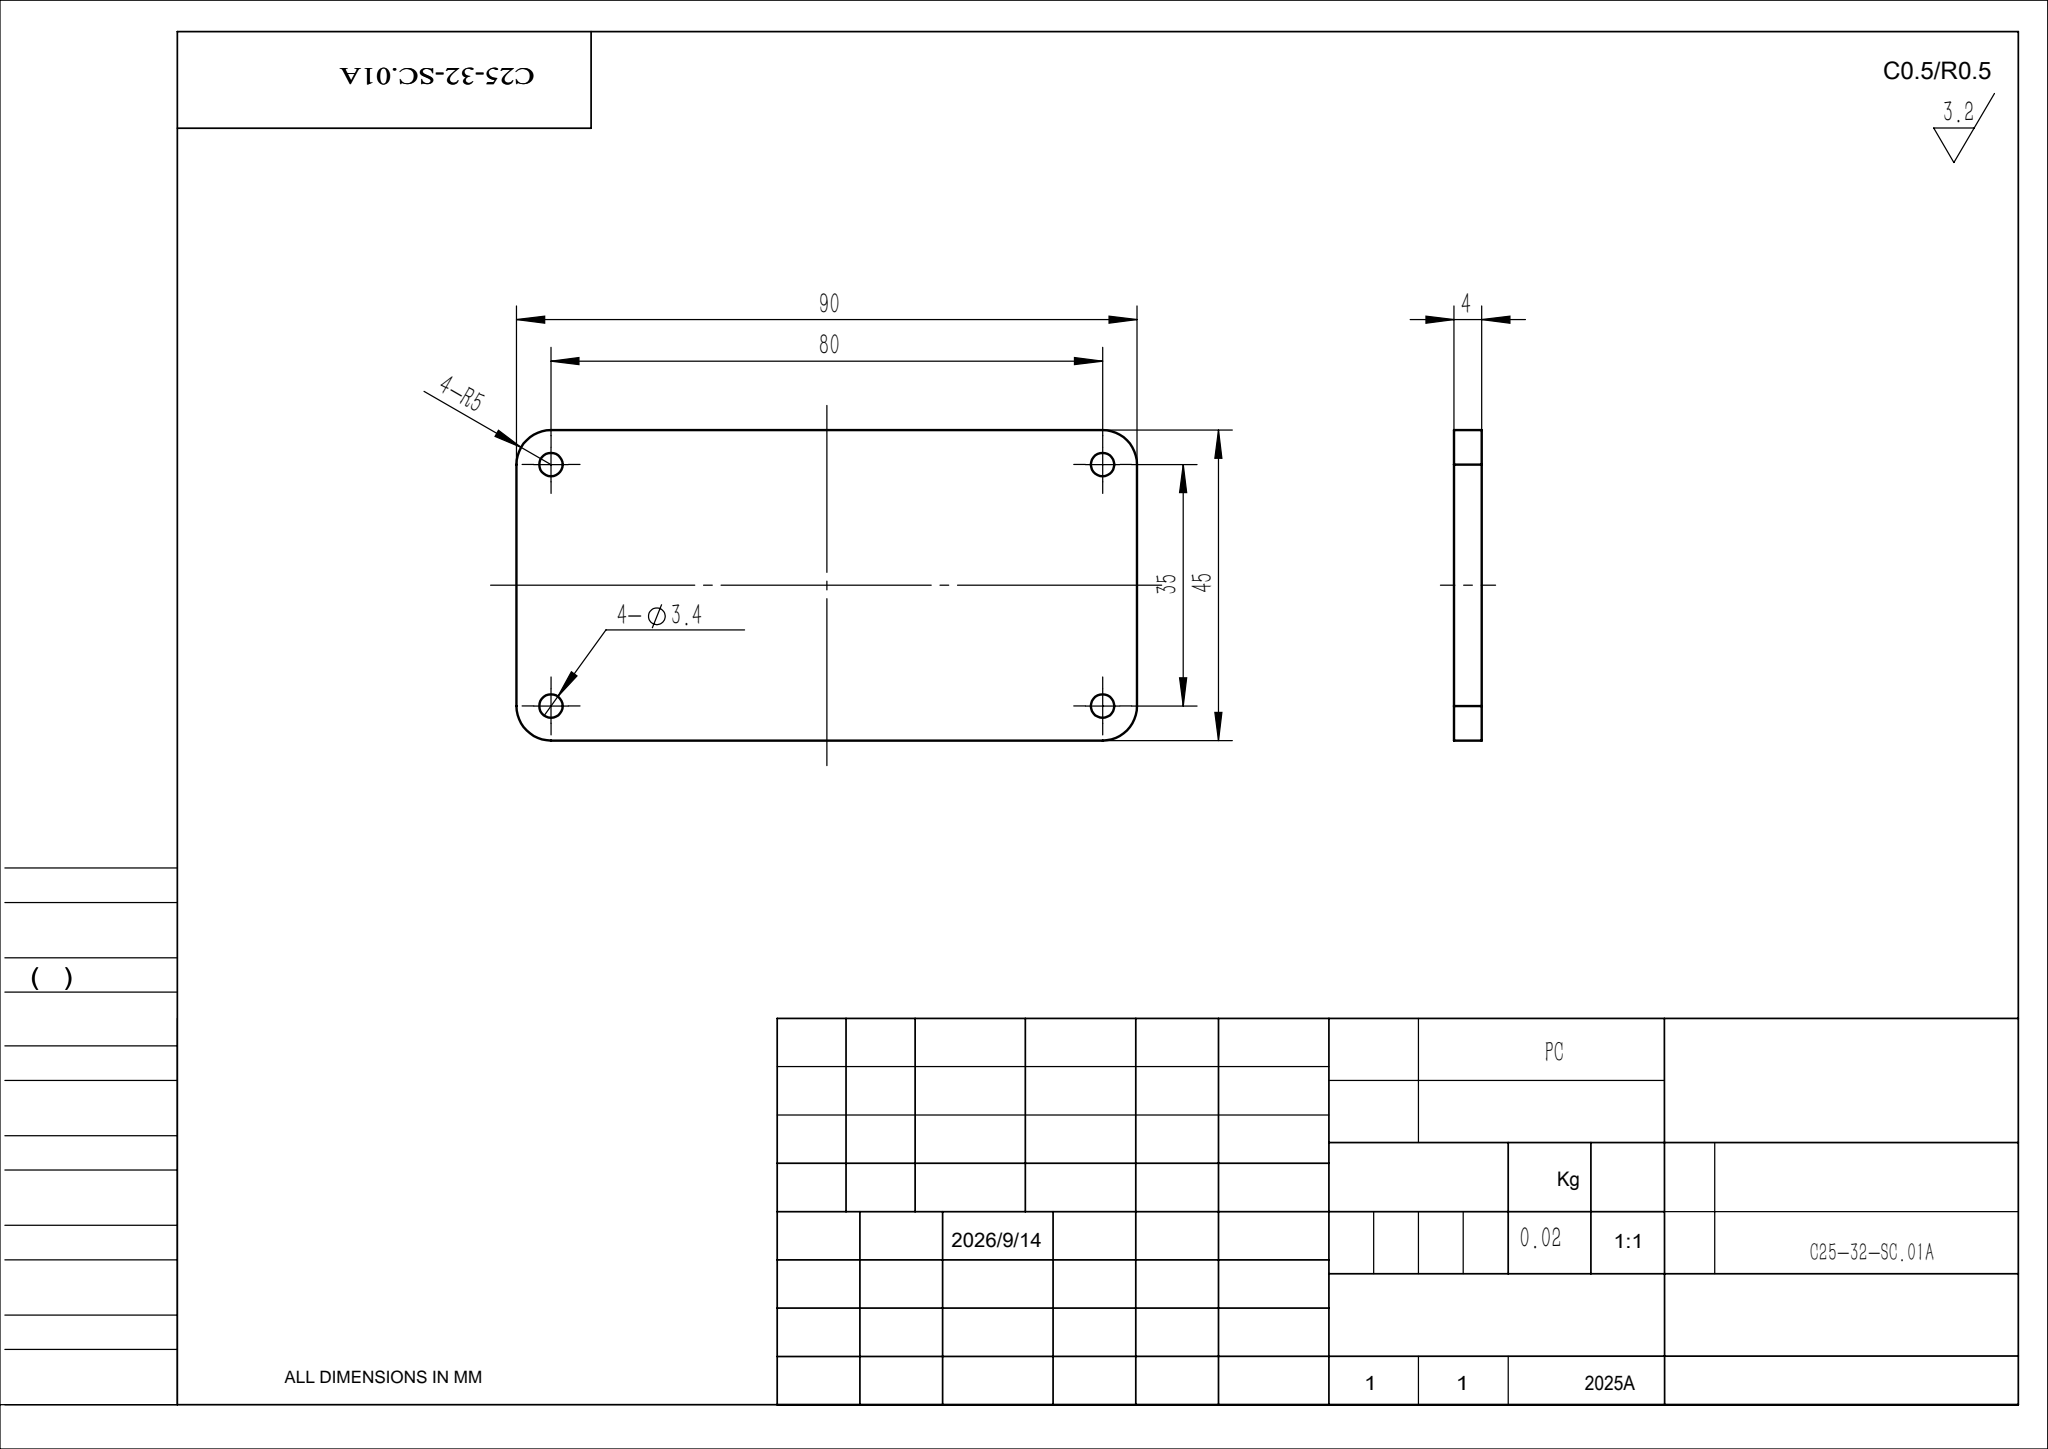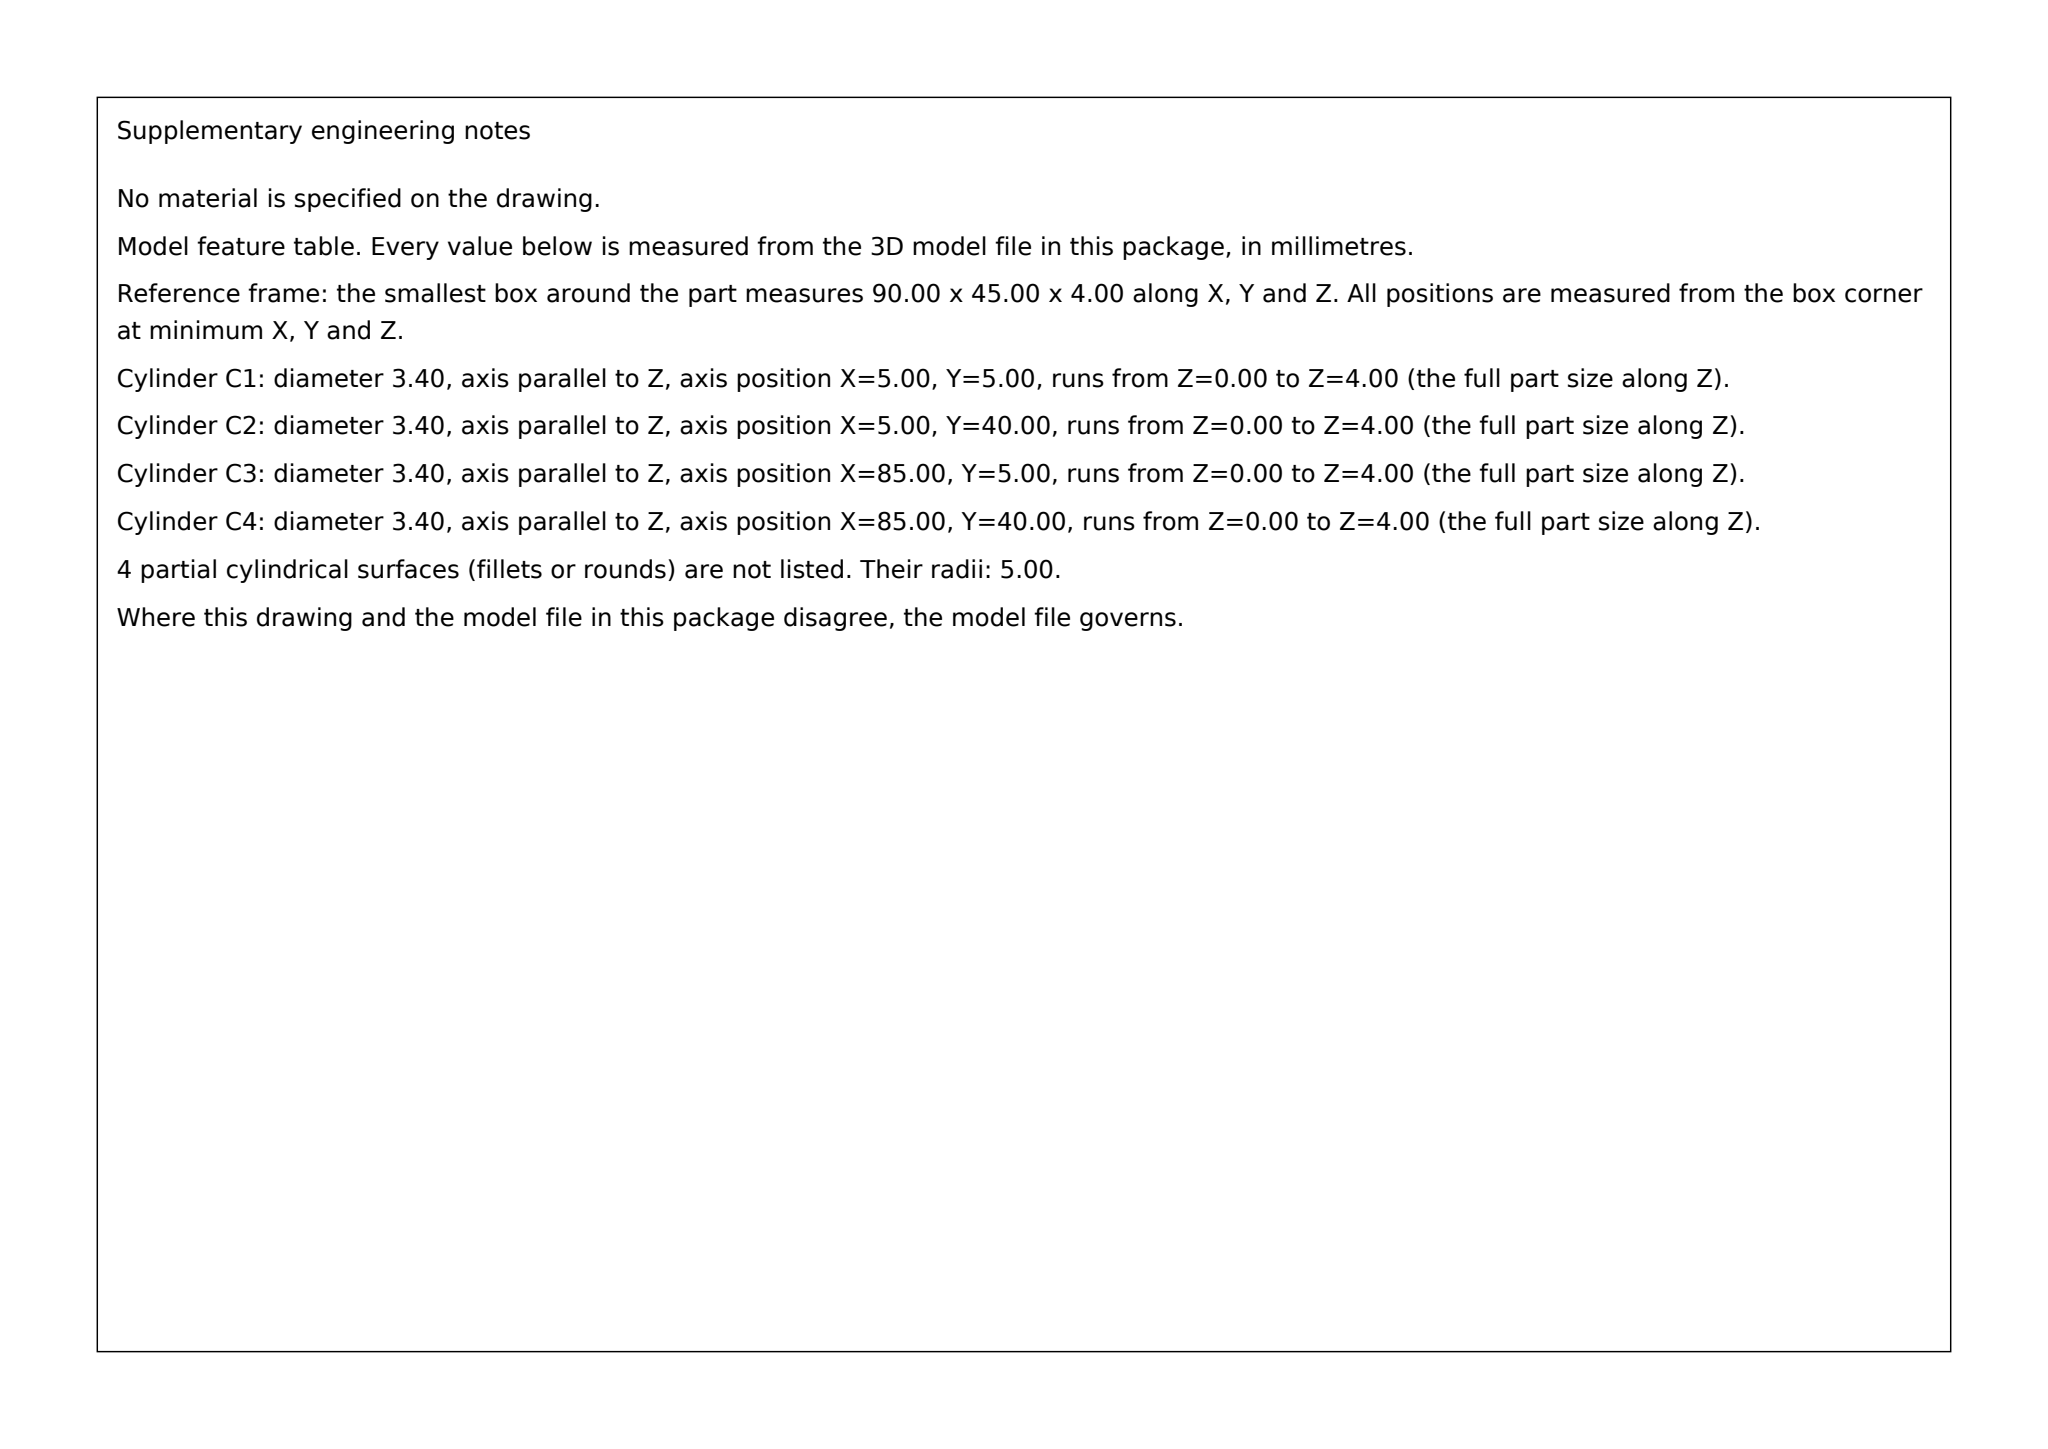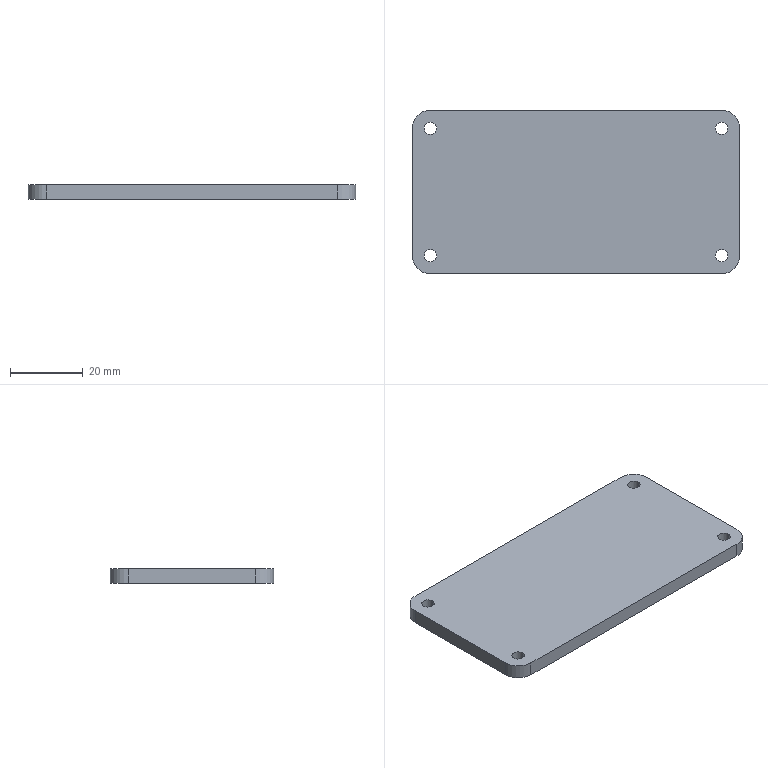Part | SolidWorks | mm | material PC | 1 solid | 18 faces | box 90 x 45 x 4 mm | volume 15969 mm3 | cylinder 12 | plane 6 | commonest cylinder face diameters 3.4 x8 10 x4
build123d program:
from build123d import *

# Parameters (mm, degrees)
BOSS_EXTRUDE1_DEPTH = 4
SKETCH2_R           = 1.7
CUT_EXTRUDE1_DEPTH  = 51.47


with BuildPart() as part:
    # Sketch1 → Boss-Extrude1 (new body)
    with BuildSketch(Plane.XY):
        with BuildLine():
            Line((40, -22.5), (-40, -22.5))
            ThreePointArc((-40, -22.5), (-43.536, -21.036), (-45, -17.5))
            Line((-45, -17.5), (-45, 17.5))
            ThreePointArc((-45, 17.5), (-43.536, 21.036), (-40, 22.5))
            Line((-40, 22.5), (40, 22.5))
            ThreePointArc((40, 22.5), (43.536, 21.036), (45, 17.5))
            Line((45, 17.5), (45, -17.5))
            ThreePointArc((45, -17.5), (43.536, -21.036), (40, -22.5))
        make_face()
    extrude(amount=BOSS_EXTRUDE1_DEPTH)

    # Sketch2 → Cut-Extrude1 (cut, through all)
    with BuildSketch(Plane.XY.offset(4)):
        with Locations((-40, 17.5)):
            Circle(SKETCH2_R)
        with Locations((-40, -17.5)):
            Circle(SKETCH2_R)
        with Locations((40, -17.5)):
            Circle(SKETCH2_R)
        with Locations((40, 17.5)):
            Circle(SKETCH2_R)
    extrude(amount=-CUT_EXTRUDE1_DEPTH, mode=Mode.SUBTRACT)


solid = part.part
STEP:
#1=CARTESIAN_POINT('',(38.3,17.5,0.));
#2=VERTEX_POINT('',#1);
#3=CARTESIAN_POINT('',(41.7,17.5,0.));
#4=VERTEX_POINT('',#3);
#5=CARTESIAN_POINT('',(40.,17.5,0.));
#6=DIRECTION('',(0.,0.,1.));
#7=DIRECTION('',(1.,0.,0.));
#8=AXIS2_PLACEMENT_3D('',#5,#6,#7);
#9=CIRCLE('',#8,1.7);
#10=EDGE_CURVE('',#2,#4,#9,.T.);
#11=ORIENTED_EDGE('',*,*,#10,.F.);
#12=CARTESIAN_POINT('',(38.3,17.5,4.));
#13=VERTEX_POINT('',#12);
#14=CARTESIAN_POINT('',(38.3,17.5,0.));
#15=DIRECTION('',(0.,0.,1.));
#16=VECTOR('',#15,1000.);
#17=LINE('',#14,#16);
#18=EDGE_CURVE('',#2,#13,#17,.T.);
#19=ORIENTED_EDGE('',*,*,#18,.T.);
#20=CARTESIAN_POINT('',(41.7,17.5,4.));
#21=VERTEX_POINT('',#20);
#22=CARTESIAN_POINT('',(40.,17.5,4.));
#23=DIRECTION('',(0.,0.,1.));
#24=DIRECTION('',(1.,0.,0.));
#25=AXIS2_PLACEMENT_3D('',#22,#23,#24);
#26=CIRCLE('',#25,1.7);
#27=EDGE_CURVE('',#13,#21,#26,.T.);
#28=ORIENTED_EDGE('',*,*,#27,.T.);
#29=CARTESIAN_POINT('',(41.7,17.5,0.));
#30=DIRECTION('',(0.,0.,1.));
#31=VECTOR('',#30,1000.);
#32=LINE('',#29,#31);
#33=EDGE_CURVE('',#4,#21,#32,.T.);
#34=ORIENTED_EDGE('',*,*,#33,.F.);
#35=EDGE_LOOP('',(#11,#19,#28,#34));
#36=FACE_OUTER_BOUND('',#35,.T.);
#37=CARTESIAN_POINT('',(40.,17.5,0.));
#38=DIRECTION('',(0.,0.,1.));
#39=DIRECTION('',(1.,0.,0.));
#40=AXIS2_PLACEMENT_3D('',#37,#38,#39);
#41=CYLINDRICAL_SURFACE('',#40,1.7);
#42=ADVANCED_FACE('',(#36),#41,.F.);
#43=CARTESIAN_POINT('',(38.3,-17.5,0.));
#44=VERTEX_POINT('',#43);
#45=CARTESIAN_POINT('',(41.7,-17.5,0.));
#46=VERTEX_POINT('',#45);
#47=CARTESIAN_POINT('',(40.,-17.5,0.));
#48=DIRECTION('',(0.,0.,1.));
#49=DIRECTION('',(1.,0.,0.));
#50=AXIS2_PLACEMENT_3D('',#47,#48,#49);
#51=CIRCLE('',#50,1.7);
#52=EDGE_CURVE('',#44,#46,#51,.T.);
#53=ORIENTED_EDGE('',*,*,#52,.F.);
#54=CARTESIAN_POINT('',(38.3,-17.5,4.));
#55=VERTEX_POINT('',#54);
#56=CARTESIAN_POINT('',(38.3,-17.5,0.));
#57=DIRECTION('',(0.,0.,1.));
#58=VECTOR('',#57,1000.);
#59=LINE('',#56,#58);
#60=EDGE_CURVE('',#44,#55,#59,.T.);
#61=ORIENTED_EDGE('',*,*,#60,.T.);
#62=CARTESIAN_POINT('',(41.7,-17.5,4.));
#63=VERTEX_POINT('',#62);
#64=CARTESIAN_POINT('',(40.,-17.5,4.));
#65=DIRECTION('',(0.,0.,1.));
#66=DIRECTION('',(1.,0.,0.));
#67=AXIS2_PLACEMENT_3D('',#64,#65,#66);
#68=CIRCLE('',#67,1.7);
#69=EDGE_CURVE('',#55,#63,#68,.T.);
#70=ORIENTED_EDGE('',*,*,#69,.T.);
#71=CARTESIAN_POINT('',(41.7,-17.5,0.));
#72=DIRECTION('',(0.,0.,1.));
#73=VECTOR('',#72,1000.);
#74=LINE('',#71,#73);
#75=EDGE_CURVE('',#46,#63,#74,.T.);
#76=ORIENTED_EDGE('',*,*,#75,.F.);
#77=EDGE_LOOP('',(#53,#61,#70,#76));
#78=FACE_OUTER_BOUND('',#77,.T.);
#79=CARTESIAN_POINT('',(40.,-17.5,0.));
#80=DIRECTION('',(0.,0.,1.));
#81=DIRECTION('',(1.,0.,0.));
#82=AXIS2_PLACEMENT_3D('',#79,#80,#81);
#83=CYLINDRICAL_SURFACE('',#82,1.7);
#84=ADVANCED_FACE('',(#78),#83,.F.);
#85=CARTESIAN_POINT('',(-41.7,-17.5,0.));
#86=VERTEX_POINT('',#85);
#87=CARTESIAN_POINT('',(-38.3,-17.5,0.));
#88=VERTEX_POINT('',#87);
#89=CARTESIAN_POINT('',(-40.,-17.5,0.));
#90=DIRECTION('',(0.,0.,1.));
#91=DIRECTION('',(1.,0.,0.));
#92=AXIS2_PLACEMENT_3D('',#89,#90,#91);
#93=CIRCLE('',#92,1.7);
#94=EDGE_CURVE('',#86,#88,#93,.T.);
#95=ORIENTED_EDGE('',*,*,#94,.F.);
#96=CARTESIAN_POINT('',(-41.7,-17.5,4.));
#97=VERTEX_POINT('',#96);
#98=CARTESIAN_POINT('',(-41.7,-17.5,0.));
#99=DIRECTION('',(0.,0.,1.));
#100=VECTOR('',#99,1000.);
#101=LINE('',#98,#100);
#102=EDGE_CURVE('',#86,#97,#101,.T.);
#103=ORIENTED_EDGE('',*,*,#102,.T.);
#104=CARTESIAN_POINT('',(-38.3,-17.5,4.));
#105=VERTEX_POINT('',#104);
#106=CARTESIAN_POINT('',(-40.,-17.5,4.));
#107=DIRECTION('',(0.,0.,1.));
#108=DIRECTION('',(1.,0.,0.));
#109=AXIS2_PLACEMENT_3D('',#106,#107,#108);
#110=CIRCLE('',#109,1.7);
#111=EDGE_CURVE('',#97,#105,#110,.T.);
#112=ORIENTED_EDGE('',*,*,#111,.T.);
#113=CARTESIAN_POINT('',(-38.3,-17.5,0.));
#114=DIRECTION('',(0.,0.,1.));
#115=VECTOR('',#114,1000.);
#116=LINE('',#113,#115);
#117=EDGE_CURVE('',#88,#105,#116,.T.);
#118=ORIENTED_EDGE('',*,*,#117,.F.);
#119=EDGE_LOOP('',(#95,#103,#112,#118));
#120=FACE_OUTER_BOUND('',#119,.T.);
#121=CARTESIAN_POINT('',(-40.,-17.5,0.));
#122=DIRECTION('',(0.,0.,1.));
#123=DIRECTION('',(1.,0.,0.));
#124=AXIS2_PLACEMENT_3D('',#121,#122,#123);
#125=CYLINDRICAL_SURFACE('',#124,1.7);
#126=ADVANCED_FACE('',(#120),#125,.F.);
#127=CARTESIAN_POINT('',(-41.7,17.5,0.));
#128=VERTEX_POINT('',#127);
#129=CARTESIAN_POINT('',(-38.3,17.5,0.));
#130=VERTEX_POINT('',#129);
#131=CARTESIAN_POINT('',(-40.,17.5,0.));
#132=DIRECTION('',(0.,0.,1.));
#133=DIRECTION('',(1.,0.,0.));
#134=AXIS2_PLACEMENT_3D('',#131,#132,#133);
#135=CIRCLE('',#134,1.7);
#136=EDGE_CURVE('',#128,#130,#135,.T.);
#137=ORIENTED_EDGE('',*,*,#136,.F.);
#138=CARTESIAN_POINT('',(-41.7,17.5,4.));
#139=VERTEX_POINT('',#138);
#140=CARTESIAN_POINT('',(-41.7,17.5,0.));
#141=DIRECTION('',(0.,0.,1.));
#142=VECTOR('',#141,1000.);
#143=LINE('',#140,#142);
#144=EDGE_CURVE('',#128,#139,#143,.T.);
#145=ORIENTED_EDGE('',*,*,#144,.T.);
#146=CARTESIAN_POINT('',(-38.3,17.5,4.));
#147=VERTEX_POINT('',#146);
#148=CARTESIAN_POINT('',(-40.,17.5,4.));
#149=DIRECTION('',(0.,0.,1.));
#150=DIRECTION('',(1.,0.,0.));
#151=AXIS2_PLACEMENT_3D('',#148,#149,#150);
#152=CIRCLE('',#151,1.7);
#153=EDGE_CURVE('',#139,#147,#152,.T.);
#154=ORIENTED_EDGE('',*,*,#153,.T.);
#155=CARTESIAN_POINT('',(-38.3,17.5,0.));
#156=DIRECTION('',(0.,0.,1.));
#157=VECTOR('',#156,1000.);
#158=LINE('',#155,#157);
#159=EDGE_CURVE('',#130,#147,#158,.T.);
#160=ORIENTED_EDGE('',*,*,#159,.F.);
#161=EDGE_LOOP('',(#137,#145,#154,#160));
#162=FACE_OUTER_BOUND('',#161,.T.);
#163=CARTESIAN_POINT('',(-40.,17.5,0.));
#164=DIRECTION('',(0.,0.,1.));
#165=DIRECTION('',(1.,0.,0.));
#166=AXIS2_PLACEMENT_3D('',#163,#164,#165);
#167=CYLINDRICAL_SURFACE('',#166,1.7);
#168=ADVANCED_FACE('',(#162),#167,.F.);
#169=CARTESIAN_POINT('',(45.,17.5,0.));
#170=VERTEX_POINT('',#169);
#171=CARTESIAN_POINT('',(40.,22.5,0.));
#172=VERTEX_POINT('',#171);
#173=CARTESIAN_POINT('',(40.,17.5,0.));
#174=DIRECTION('',(0.,0.,1.));
#175=DIRECTION('',(1.,0.,0.));
#176=AXIS2_PLACEMENT_3D('',#173,#174,#175);
#177=CIRCLE('',#176,5.);
#178=EDGE_CURVE('',#170,#172,#177,.T.);
#179=ORIENTED_EDGE('',*,*,#178,.T.);
#180=CARTESIAN_POINT('',(40.,22.5,4.));
#181=VERTEX_POINT('',#180);
#182=CARTESIAN_POINT('',(40.,22.5,4.));
#183=DIRECTION('',(0.,0.,-1.));
#184=VECTOR('',#183,1000.);
#185=LINE('',#182,#184);
#186=EDGE_CURVE('',#181,#172,#185,.T.);
#187=ORIENTED_EDGE('',*,*,#186,.F.);
#188=CARTESIAN_POINT('',(45.,17.5,4.));
#189=VERTEX_POINT('',#188);
#190=CARTESIAN_POINT('',(40.,17.5,4.));
#191=DIRECTION('',(0.,0.,1.));
#192=DIRECTION('',(1.,0.,0.));
#193=AXIS2_PLACEMENT_3D('',#190,#191,#192);
#194=CIRCLE('',#193,5.);
#195=EDGE_CURVE('',#189,#181,#194,.T.);
#196=ORIENTED_EDGE('',*,*,#195,.F.);
#197=CARTESIAN_POINT('',(45.,17.5,4.));
#198=DIRECTION('',(0.,0.,-1.));
#199=VECTOR('',#198,1000.);
#200=LINE('',#197,#199);
#201=EDGE_CURVE('',#189,#170,#200,.T.);
#202=ORIENTED_EDGE('',*,*,#201,.T.);
#203=EDGE_LOOP('',(#179,#187,#196,#202));
#204=FACE_OUTER_BOUND('',#203,.T.);
#205=CARTESIAN_POINT('',(40.,17.5,4.));
#206=DIRECTION('',(0.,0.,-1.));
#207=DIRECTION('',(-1.,0.,0.));
#208=AXIS2_PLACEMENT_3D('',#205,#206,#207);
#209=CYLINDRICAL_SURFACE('',#208,5.);
#210=ADVANCED_FACE('',(#204),#209,.T.);
#211=CARTESIAN_POINT('',(-40.,22.5,0.));
#212=VERTEX_POINT('',#211);
#213=CARTESIAN_POINT('',(40.,22.5,0.));
#214=DIRECTION('',(-1.,-0.,0.));
#215=VECTOR('',#214,1000.);
#216=LINE('',#213,#215);
#217=EDGE_CURVE('',#172,#212,#216,.T.);
#218=ORIENTED_EDGE('',*,*,#217,.T.);
#219=CARTESIAN_POINT('',(-40.,22.5,4.));
#220=VERTEX_POINT('',#219);
#221=CARTESIAN_POINT('',(-40.,22.5,4.));
#222=DIRECTION('',(0.,0.,-1.));
#223=VECTOR('',#222,1000.);
#224=LINE('',#221,#223);
#225=EDGE_CURVE('',#220,#212,#224,.T.);
#226=ORIENTED_EDGE('',*,*,#225,.F.);
#227=CARTESIAN_POINT('',(40.,22.5,4.));
#228=DIRECTION('',(-1.,-0.,0.));
#229=VECTOR('',#228,1000.);
#230=LINE('',#227,#229);
#231=EDGE_CURVE('',#181,#220,#230,.T.);
#232=ORIENTED_EDGE('',*,*,#231,.F.);
#233=ORIENTED_EDGE('',*,*,#186,.T.);
#234=EDGE_LOOP('',(#218,#226,#232,#233));
#235=FACE_OUTER_BOUND('',#234,.T.);
#236=CARTESIAN_POINT('',(40.,22.5,4.));
#237=DIRECTION('',(0.,-1.,0.));
#238=DIRECTION('',(1.,0.,0.));
#239=AXIS2_PLACEMENT_3D('',#236,#237,#238);
#240=PLANE('',#239);
#241=ADVANCED_FACE('',(#235),#240,.F.);
#242=CARTESIAN_POINT('',(-45.,17.5,0.));
#243=VERTEX_POINT('',#242);
#244=CARTESIAN_POINT('',(-40.,17.5,0.));
#245=DIRECTION('',(0.,0.,1.));
#246=DIRECTION('',(-1.,0.,0.));
#247=AXIS2_PLACEMENT_3D('',#244,#245,#246);
#248=CIRCLE('',#247,5.);
#249=EDGE_CURVE('',#212,#243,#248,.T.);
#250=ORIENTED_EDGE('',*,*,#249,.T.);
#251=CARTESIAN_POINT('',(-45.,17.5,4.));
#252=VERTEX_POINT('',#251);
#253=CARTESIAN_POINT('',(-45.,17.5,4.));
#254=DIRECTION('',(0.,0.,-1.));
#255=VECTOR('',#254,1000.);
#256=LINE('',#253,#255);
#257=EDGE_CURVE('',#252,#243,#256,.T.);
#258=ORIENTED_EDGE('',*,*,#257,.F.);
#259=CARTESIAN_POINT('',(-40.,17.5,4.));
#260=DIRECTION('',(0.,0.,1.));
#261=DIRECTION('',(-1.,0.,0.));
#262=AXIS2_PLACEMENT_3D('',#259,#260,#261);
#263=CIRCLE('',#262,5.);
#264=EDGE_CURVE('',#220,#252,#263,.T.);
#265=ORIENTED_EDGE('',*,*,#264,.F.);
#266=ORIENTED_EDGE('',*,*,#225,.T.);
#267=EDGE_LOOP('',(#250,#258,#265,#266));
#268=FACE_OUTER_BOUND('',#267,.T.);
#269=CARTESIAN_POINT('',(-40.,17.5,4.));
#270=DIRECTION('',(0.,0.,-1.));
#271=DIRECTION('',(-1.,0.,0.));
#272=AXIS2_PLACEMENT_3D('',#269,#270,#271);
#273=CYLINDRICAL_SURFACE('',#272,5.);
#274=ADVANCED_FACE('',(#268),#273,.T.);
#275=CARTESIAN_POINT('',(-45.,-17.5,0.));
#276=VERTEX_POINT('',#275);
#277=CARTESIAN_POINT('',(-45.,-17.5,0.));
#278=DIRECTION('',(0.,-1.,0.));
#279=VECTOR('',#278,1000.);
#280=LINE('',#277,#279);
#281=EDGE_CURVE('',#243,#276,#280,.T.);
#282=ORIENTED_EDGE('',*,*,#281,.T.);
#283=CARTESIAN_POINT('',(-45.,-17.5,4.));
#284=VERTEX_POINT('',#283);
#285=CARTESIAN_POINT('',(-45.,-17.5,4.));
#286=DIRECTION('',(0.,0.,-1.));
#287=VECTOR('',#286,1000.);
#288=LINE('',#285,#287);
#289=EDGE_CURVE('',#284,#276,#288,.T.);
#290=ORIENTED_EDGE('',*,*,#289,.F.);
#291=CARTESIAN_POINT('',(-45.,-17.5,4.));
#292=DIRECTION('',(0.,-1.,0.));
#293=VECTOR('',#292,1000.);
#294=LINE('',#291,#293);
#295=EDGE_CURVE('',#252,#284,#294,.T.);
#296=ORIENTED_EDGE('',*,*,#295,.F.);
#297=ORIENTED_EDGE('',*,*,#257,.T.);
#298=EDGE_LOOP('',(#282,#290,#296,#297));
#299=FACE_OUTER_BOUND('',#298,.T.);
#300=CARTESIAN_POINT('',(-45.,-17.5,4.));
#301=DIRECTION('',(1.,0.,0.));
#302=DIRECTION('',(0.,0.,-1.));
#303=AXIS2_PLACEMENT_3D('',#300,#301,#302);
#304=PLANE('',#303);
#305=ADVANCED_FACE('',(#299),#304,.F.);
#306=CARTESIAN_POINT('',(-40.,-22.5,0.));
#307=VERTEX_POINT('',#306);
#308=CARTESIAN_POINT('',(-40.,-17.5,0.));
#309=DIRECTION('',(0.,0.,1.));
#310=DIRECTION('',(-1.,0.,0.));
#311=AXIS2_PLACEMENT_3D('',#308,#309,#310);
#312=CIRCLE('',#311,5.);
#313=EDGE_CURVE('',#276,#307,#312,.T.);
#314=ORIENTED_EDGE('',*,*,#313,.T.);
#315=CARTESIAN_POINT('',(-40.,-22.5,4.));
#316=VERTEX_POINT('',#315);
#317=CARTESIAN_POINT('',(-40.,-22.5,4.));
#318=DIRECTION('',(0.,0.,-1.));
#319=VECTOR('',#318,1000.);
#320=LINE('',#317,#319);
#321=EDGE_CURVE('',#316,#307,#320,.T.);
#322=ORIENTED_EDGE('',*,*,#321,.F.);
#323=CARTESIAN_POINT('',(-40.,-17.5,4.));
#324=DIRECTION('',(0.,0.,1.));
#325=DIRECTION('',(-1.,0.,0.));
#326=AXIS2_PLACEMENT_3D('',#323,#324,#325);
#327=CIRCLE('',#326,5.);
#328=EDGE_CURVE('',#284,#316,#327,.T.);
#329=ORIENTED_EDGE('',*,*,#328,.F.);
#330=ORIENTED_EDGE('',*,*,#289,.T.);
#331=EDGE_LOOP('',(#314,#322,#329,#330));
#332=FACE_OUTER_BOUND('',#331,.T.);
#333=CARTESIAN_POINT('',(-40.,-17.5,4.));
#334=DIRECTION('',(0.,0.,-1.));
#335=DIRECTION('',(-1.,0.,0.));
#336=AXIS2_PLACEMENT_3D('',#333,#334,#335);
#337=CYLINDRICAL_SURFACE('',#336,5.);
#338=ADVANCED_FACE('',(#332),#337,.T.);
#339=CARTESIAN_POINT('',(40.,-22.5,0.));
#340=VERTEX_POINT('',#339);
#341=CARTESIAN_POINT('',(40.,-22.5,0.));
#342=DIRECTION('',(1.,0.,0.));
#343=VECTOR('',#342,1000.);
#344=LINE('',#341,#343);
#345=EDGE_CURVE('',#307,#340,#344,.T.);
#346=ORIENTED_EDGE('',*,*,#345,.T.);
#347=CARTESIAN_POINT('',(40.,-22.5,4.));
#348=VERTEX_POINT('',#347);
#349=CARTESIAN_POINT('',(40.,-22.5,4.));
#350=DIRECTION('',(0.,0.,-1.));
#351=VECTOR('',#350,1000.);
#352=LINE('',#349,#351);
#353=EDGE_CURVE('',#348,#340,#352,.T.);
#354=ORIENTED_EDGE('',*,*,#353,.F.);
#355=CARTESIAN_POINT('',(40.,-22.5,4.));
#356=DIRECTION('',(1.,0.,0.));
#357=VECTOR('',#356,1000.);
#358=LINE('',#355,#357);
#359=EDGE_CURVE('',#316,#348,#358,.T.);
#360=ORIENTED_EDGE('',*,*,#359,.F.);
#361=ORIENTED_EDGE('',*,*,#321,.T.);
#362=EDGE_LOOP('',(#346,#354,#360,#361));
#363=FACE_OUTER_BOUND('',#362,.T.);
#364=CARTESIAN_POINT('',(40.,-22.5,4.));
#365=DIRECTION('',(-0.,1.,0.));
#366=DIRECTION('',(-1.,-0.,0.));
#367=AXIS2_PLACEMENT_3D('',#364,#365,#366);
#368=PLANE('',#367);
#369=ADVANCED_FACE('',(#363),#368,.F.);
#370=CARTESIAN_POINT('',(45.,-17.5,0.));
#371=VERTEX_POINT('',#370);
#372=CARTESIAN_POINT('',(40.,-17.5,0.));
#373=DIRECTION('',(0.,0.,1.));
#374=DIRECTION('',(-1.,0.,0.));
#375=AXIS2_PLACEMENT_3D('',#372,#373,#374);
#376=CIRCLE('',#375,5.);
#377=EDGE_CURVE('',#340,#371,#376,.T.);
#378=ORIENTED_EDGE('',*,*,#377,.T.);
#379=CARTESIAN_POINT('',(45.,-17.5,4.));
#380=VERTEX_POINT('',#379);
#381=CARTESIAN_POINT('',(45.,-17.5,4.));
#382=DIRECTION('',(0.,0.,-1.));
#383=VECTOR('',#382,1000.);
#384=LINE('',#381,#383);
#385=EDGE_CURVE('',#380,#371,#384,.T.);
#386=ORIENTED_EDGE('',*,*,#385,.F.);
#387=CARTESIAN_POINT('',(40.,-17.5,4.));
#388=DIRECTION('',(0.,0.,1.));
#389=DIRECTION('',(-1.,0.,0.));
#390=AXIS2_PLACEMENT_3D('',#387,#388,#389);
#391=CIRCLE('',#390,5.);
#392=EDGE_CURVE('',#348,#380,#391,.T.);
#393=ORIENTED_EDGE('',*,*,#392,.F.);
#394=ORIENTED_EDGE('',*,*,#353,.T.);
#395=EDGE_LOOP('',(#378,#386,#393,#394));
#396=FACE_OUTER_BOUND('',#395,.T.);
#397=CARTESIAN_POINT('',(40.,-17.5,4.));
#398=DIRECTION('',(0.,0.,-1.));
#399=DIRECTION('',(-1.,0.,0.));
#400=AXIS2_PLACEMENT_3D('',#397,#398,#399);
#401=CYLINDRICAL_SURFACE('',#400,5.);
#402=ADVANCED_FACE('',(#396),#401,.T.);
#403=CARTESIAN_POINT('',(45.,-17.5,0.));
#404=DIRECTION('',(0.,1.,0.));
#405=VECTOR('',#404,1000.);
#406=LINE('',#403,#405);
#407=EDGE_CURVE('',#371,#170,#406,.T.);
#408=ORIENTED_EDGE('',*,*,#407,.T.);
#409=ORIENTED_EDGE('',*,*,#201,.F.);
#410=CARTESIAN_POINT('',(45.,-17.5,4.));
#411=DIRECTION('',(0.,1.,0.));
#412=VECTOR('',#411,1000.);
#413=LINE('',#410,#412);
#414=EDGE_CURVE('',#380,#189,#413,.T.);
#415=ORIENTED_EDGE('',*,*,#414,.F.);
#416=ORIENTED_EDGE('',*,*,#385,.T.);
#417=EDGE_LOOP('',(#408,#409,#415,#416));
#418=FACE_OUTER_BOUND('',#417,.T.);
#419=CARTESIAN_POINT('',(45.,-17.5,4.));
#420=DIRECTION('',(-1.,0.,0.));
#421=DIRECTION('',(0.,0.,1.));
#422=AXIS2_PLACEMENT_3D('',#419,#420,#421);
#423=PLANE('',#422);
#424=ADVANCED_FACE('',(#418),#423,.F.);
#425=CARTESIAN_POINT('',(40.,17.5,4.));
#426=DIRECTION('',(0.,0.,1.));
#427=DIRECTION('',(1.,0.,0.));
#428=AXIS2_PLACEMENT_3D('',#425,#426,#427);
#429=CIRCLE('',#428,1.7);
#430=EDGE_CURVE('',#21,#13,#429,.T.);
#431=ORIENTED_EDGE('',*,*,#430,.F.);
#432=ORIENTED_EDGE('',*,*,#27,.F.);
#433=EDGE_LOOP('',(#431,#432));
#434=FACE_BOUND('',#433,.T.);
#435=CARTESIAN_POINT('',(40.,-17.5,4.));
#436=DIRECTION('',(0.,0.,1.));
#437=DIRECTION('',(1.,0.,0.));
#438=AXIS2_PLACEMENT_3D('',#435,#436,#437);
#439=CIRCLE('',#438,1.7);
#440=EDGE_CURVE('',#63,#55,#439,.T.);
#441=ORIENTED_EDGE('',*,*,#440,.F.);
#442=ORIENTED_EDGE('',*,*,#69,.F.);
#443=EDGE_LOOP('',(#441,#442));
#444=FACE_BOUND('',#443,.T.);
#445=CARTESIAN_POINT('',(-40.,-17.5,4.));
#446=DIRECTION('',(0.,0.,1.));
#447=DIRECTION('',(1.,0.,0.));
#448=AXIS2_PLACEMENT_3D('',#445,#446,#447);
#449=CIRCLE('',#448,1.7);
#450=EDGE_CURVE('',#105,#97,#449,.T.);
#451=ORIENTED_EDGE('',*,*,#450,.F.);
#452=ORIENTED_EDGE('',*,*,#111,.F.);
#453=EDGE_LOOP('',(#451,#452));
#454=FACE_BOUND('',#453,.T.);
#455=CARTESIAN_POINT('',(-40.,17.5,4.));
#456=DIRECTION('',(0.,0.,1.));
#457=DIRECTION('',(1.,0.,0.));
#458=AXIS2_PLACEMENT_3D('',#455,#456,#457);
#459=CIRCLE('',#458,1.7);
#460=EDGE_CURVE('',#147,#139,#459,.T.);
#461=ORIENTED_EDGE('',*,*,#460,.F.);
#462=ORIENTED_EDGE('',*,*,#153,.F.);
#463=EDGE_LOOP('',(#461,#462));
#464=FACE_BOUND('',#463,.T.);
#465=ORIENTED_EDGE('',*,*,#195,.T.);
#466=ORIENTED_EDGE('',*,*,#231,.T.);
#467=ORIENTED_EDGE('',*,*,#264,.T.);
#468=ORIENTED_EDGE('',*,*,#295,.T.);
#469=ORIENTED_EDGE('',*,*,#328,.T.);
#470=ORIENTED_EDGE('',*,*,#359,.T.);
#471=ORIENTED_EDGE('',*,*,#392,.T.);
#472=ORIENTED_EDGE('',*,*,#414,.T.);
#473=EDGE_LOOP('',(#465,#466,#467,#468,#469,#470,#471,#472));
#474=FACE_OUTER_BOUND('',#473,.T.);
#475=CARTESIAN_POINT('',(40.,17.5,4.));
#476=DIRECTION('',(0.,0.,1.));
#477=DIRECTION('',(1.,0.,0.));
#478=AXIS2_PLACEMENT_3D('',#475,#476,#477);
#479=PLANE('',#478);
#480=ADVANCED_FACE('',(#434,#444,#454,#464,#474),#479,.T.);
#481=CARTESIAN_POINT('',(40.,17.5,0.));
#482=DIRECTION('',(0.,0.,1.));
#483=DIRECTION('',(1.,0.,0.));
#484=AXIS2_PLACEMENT_3D('',#481,#482,#483);
#485=CIRCLE('',#484,1.7);
#486=EDGE_CURVE('',#4,#2,#485,.T.);
#487=ORIENTED_EDGE('',*,*,#486,.T.);
#488=ORIENTED_EDGE('',*,*,#10,.T.);
#489=EDGE_LOOP('',(#487,#488));
#490=FACE_BOUND('',#489,.T.);
#491=CARTESIAN_POINT('',(40.,-17.5,0.));
#492=DIRECTION('',(0.,0.,1.));
#493=DIRECTION('',(1.,0.,0.));
#494=AXIS2_PLACEMENT_3D('',#491,#492,#493);
#495=CIRCLE('',#494,1.7);
#496=EDGE_CURVE('',#46,#44,#495,.T.);
#497=ORIENTED_EDGE('',*,*,#496,.T.);
#498=ORIENTED_EDGE('',*,*,#52,.T.);
#499=EDGE_LOOP('',(#497,#498));
#500=FACE_BOUND('',#499,.T.);
#501=CARTESIAN_POINT('',(-40.,-17.5,0.));
#502=DIRECTION('',(0.,0.,1.));
#503=DIRECTION('',(1.,0.,0.));
#504=AXIS2_PLACEMENT_3D('',#501,#502,#503);
#505=CIRCLE('',#504,1.7);
#506=EDGE_CURVE('',#88,#86,#505,.T.);
#507=ORIENTED_EDGE('',*,*,#506,.T.);
#508=ORIENTED_EDGE('',*,*,#94,.T.);
#509=EDGE_LOOP('',(#507,#508));
#510=FACE_BOUND('',#509,.T.);
#511=CARTESIAN_POINT('',(-40.,17.5,0.));
#512=DIRECTION('',(0.,0.,1.));
#513=DIRECTION('',(1.,0.,0.));
#514=AXIS2_PLACEMENT_3D('',#511,#512,#513);
#515=CIRCLE('',#514,1.7);
#516=EDGE_CURVE('',#130,#128,#515,.T.);
#517=ORIENTED_EDGE('',*,*,#516,.T.);
#518=ORIENTED_EDGE('',*,*,#136,.T.);
#519=EDGE_LOOP('',(#517,#518));
#520=FACE_BOUND('',#519,.T.);
#521=ORIENTED_EDGE('',*,*,#178,.F.);
#522=ORIENTED_EDGE('',*,*,#407,.F.);
#523=ORIENTED_EDGE('',*,*,#377,.F.);
#524=ORIENTED_EDGE('',*,*,#345,.F.);
#525=ORIENTED_EDGE('',*,*,#313,.F.);
#526=ORIENTED_EDGE('',*,*,#281,.F.);
#527=ORIENTED_EDGE('',*,*,#249,.F.);
#528=ORIENTED_EDGE('',*,*,#217,.F.);
#529=EDGE_LOOP('',(#521,#522,#523,#524,#525,#526,#527,#528));
#530=FACE_OUTER_BOUND('',#529,.T.);
#531=CARTESIAN_POINT('',(40.,17.5,0.));
#532=DIRECTION('',(0.,0.,1.));
#533=DIRECTION('',(1.,0.,0.));
#534=AXIS2_PLACEMENT_3D('',#531,#532,#533);
#535=PLANE('',#534);
#536=ADVANCED_FACE('',(#490,#500,#510,#520,#530),#535,.F.);
#537=ORIENTED_EDGE('',*,*,#144,.F.);
#538=ORIENTED_EDGE('',*,*,#516,.F.);
#539=ORIENTED_EDGE('',*,*,#159,.T.);
#540=ORIENTED_EDGE('',*,*,#460,.T.);
#541=EDGE_LOOP('',(#537,#538,#539,#540));
#542=FACE_OUTER_BOUND('',#541,.T.);
#543=CARTESIAN_POINT('',(-40.,17.5,0.));
#544=DIRECTION('',(0.,0.,1.));
#545=DIRECTION('',(1.,0.,0.));
#546=AXIS2_PLACEMENT_3D('',#543,#544,#545);
#547=CYLINDRICAL_SURFACE('',#546,1.7);
#548=ADVANCED_FACE('',(#542),#547,.F.);
#549=ORIENTED_EDGE('',*,*,#102,.F.);
#550=ORIENTED_EDGE('',*,*,#506,.F.);
#551=ORIENTED_EDGE('',*,*,#117,.T.);
#552=ORIENTED_EDGE('',*,*,#450,.T.);
#553=EDGE_LOOP('',(#549,#550,#551,#552));
#554=FACE_OUTER_BOUND('',#553,.T.);
#555=CARTESIAN_POINT('',(-40.,-17.5,0.));
#556=DIRECTION('',(0.,0.,1.));
#557=DIRECTION('',(1.,0.,0.));
#558=AXIS2_PLACEMENT_3D('',#555,#556,#557);
#559=CYLINDRICAL_SURFACE('',#558,1.7);
#560=ADVANCED_FACE('',(#554),#559,.F.);
#561=ORIENTED_EDGE('',*,*,#60,.F.);
#562=ORIENTED_EDGE('',*,*,#496,.F.);
#563=ORIENTED_EDGE('',*,*,#75,.T.);
#564=ORIENTED_EDGE('',*,*,#440,.T.);
#565=EDGE_LOOP('',(#561,#562,#563,#564));
#566=FACE_OUTER_BOUND('',#565,.T.);
#567=CARTESIAN_POINT('',(40.,-17.5,0.));
#568=DIRECTION('',(0.,0.,1.));
#569=DIRECTION('',(1.,0.,0.));
#570=AXIS2_PLACEMENT_3D('',#567,#568,#569);
#571=CYLINDRICAL_SURFACE('',#570,1.7);
#572=ADVANCED_FACE('',(#566),#571,.F.);
#573=ORIENTED_EDGE('',*,*,#18,.F.);
#574=ORIENTED_EDGE('',*,*,#486,.F.);
#575=ORIENTED_EDGE('',*,*,#33,.T.);
#576=ORIENTED_EDGE('',*,*,#430,.T.);
#577=EDGE_LOOP('',(#573,#574,#575,#576));
#578=FACE_OUTER_BOUND('',#577,.T.);
#579=CARTESIAN_POINT('',(40.,17.5,0.));
#580=DIRECTION('',(0.,0.,1.));
#581=DIRECTION('',(1.,0.,0.));
#582=AXIS2_PLACEMENT_3D('',#579,#580,#581);
#583=CYLINDRICAL_SURFACE('',#582,1.7);
#584=ADVANCED_FACE('',(#578),#583,.F.);
#585=CLOSED_SHELL('',(#42,#84,#126,#168,#210,#241,#274,#305,#338,#369,#402,#424,#480,#536,#548,#560,#572,#584));
#586=MANIFOLD_SOLID_BREP('',#585);
#587=CARTESIAN_POINT('',(0.,0.,0.));
#588=DIRECTION('',(0.,0.,1.));
#589=DIRECTION('',(1.,0.,0.));
#590=AXIS2_PLACEMENT_3D('',#587,#588,#589);
#591=(LENGTH_UNIT()NAMED_UNIT(*)SI_UNIT(.MILLI.,.METRE.));
#592=UNCERTAINTY_MEASURE_WITH_UNIT(LENGTH_MEASURE(0.00001),#591,'','');
#593=(NAMED_UNIT(*)PLANE_ANGLE_UNIT()SI_UNIT($,.RADIAN.));
#594=(NAMED_UNIT(*)SI_UNIT($,.STERADIAN.)SOLID_ANGLE_UNIT());
#595=(GEOMETRIC_REPRESENTATION_CONTEXT(3)GLOBAL_UNCERTAINTY_ASSIGNED_CONTEXT((#592))GLOBAL_UNIT_ASSIGNED_CONTEXT((#591,#593,#594))REPRESENTATION_CONTEXT('',''));
#596=ADVANCED_BREP_SHAPE_REPRESENTATION('',(#586,#590),#595);